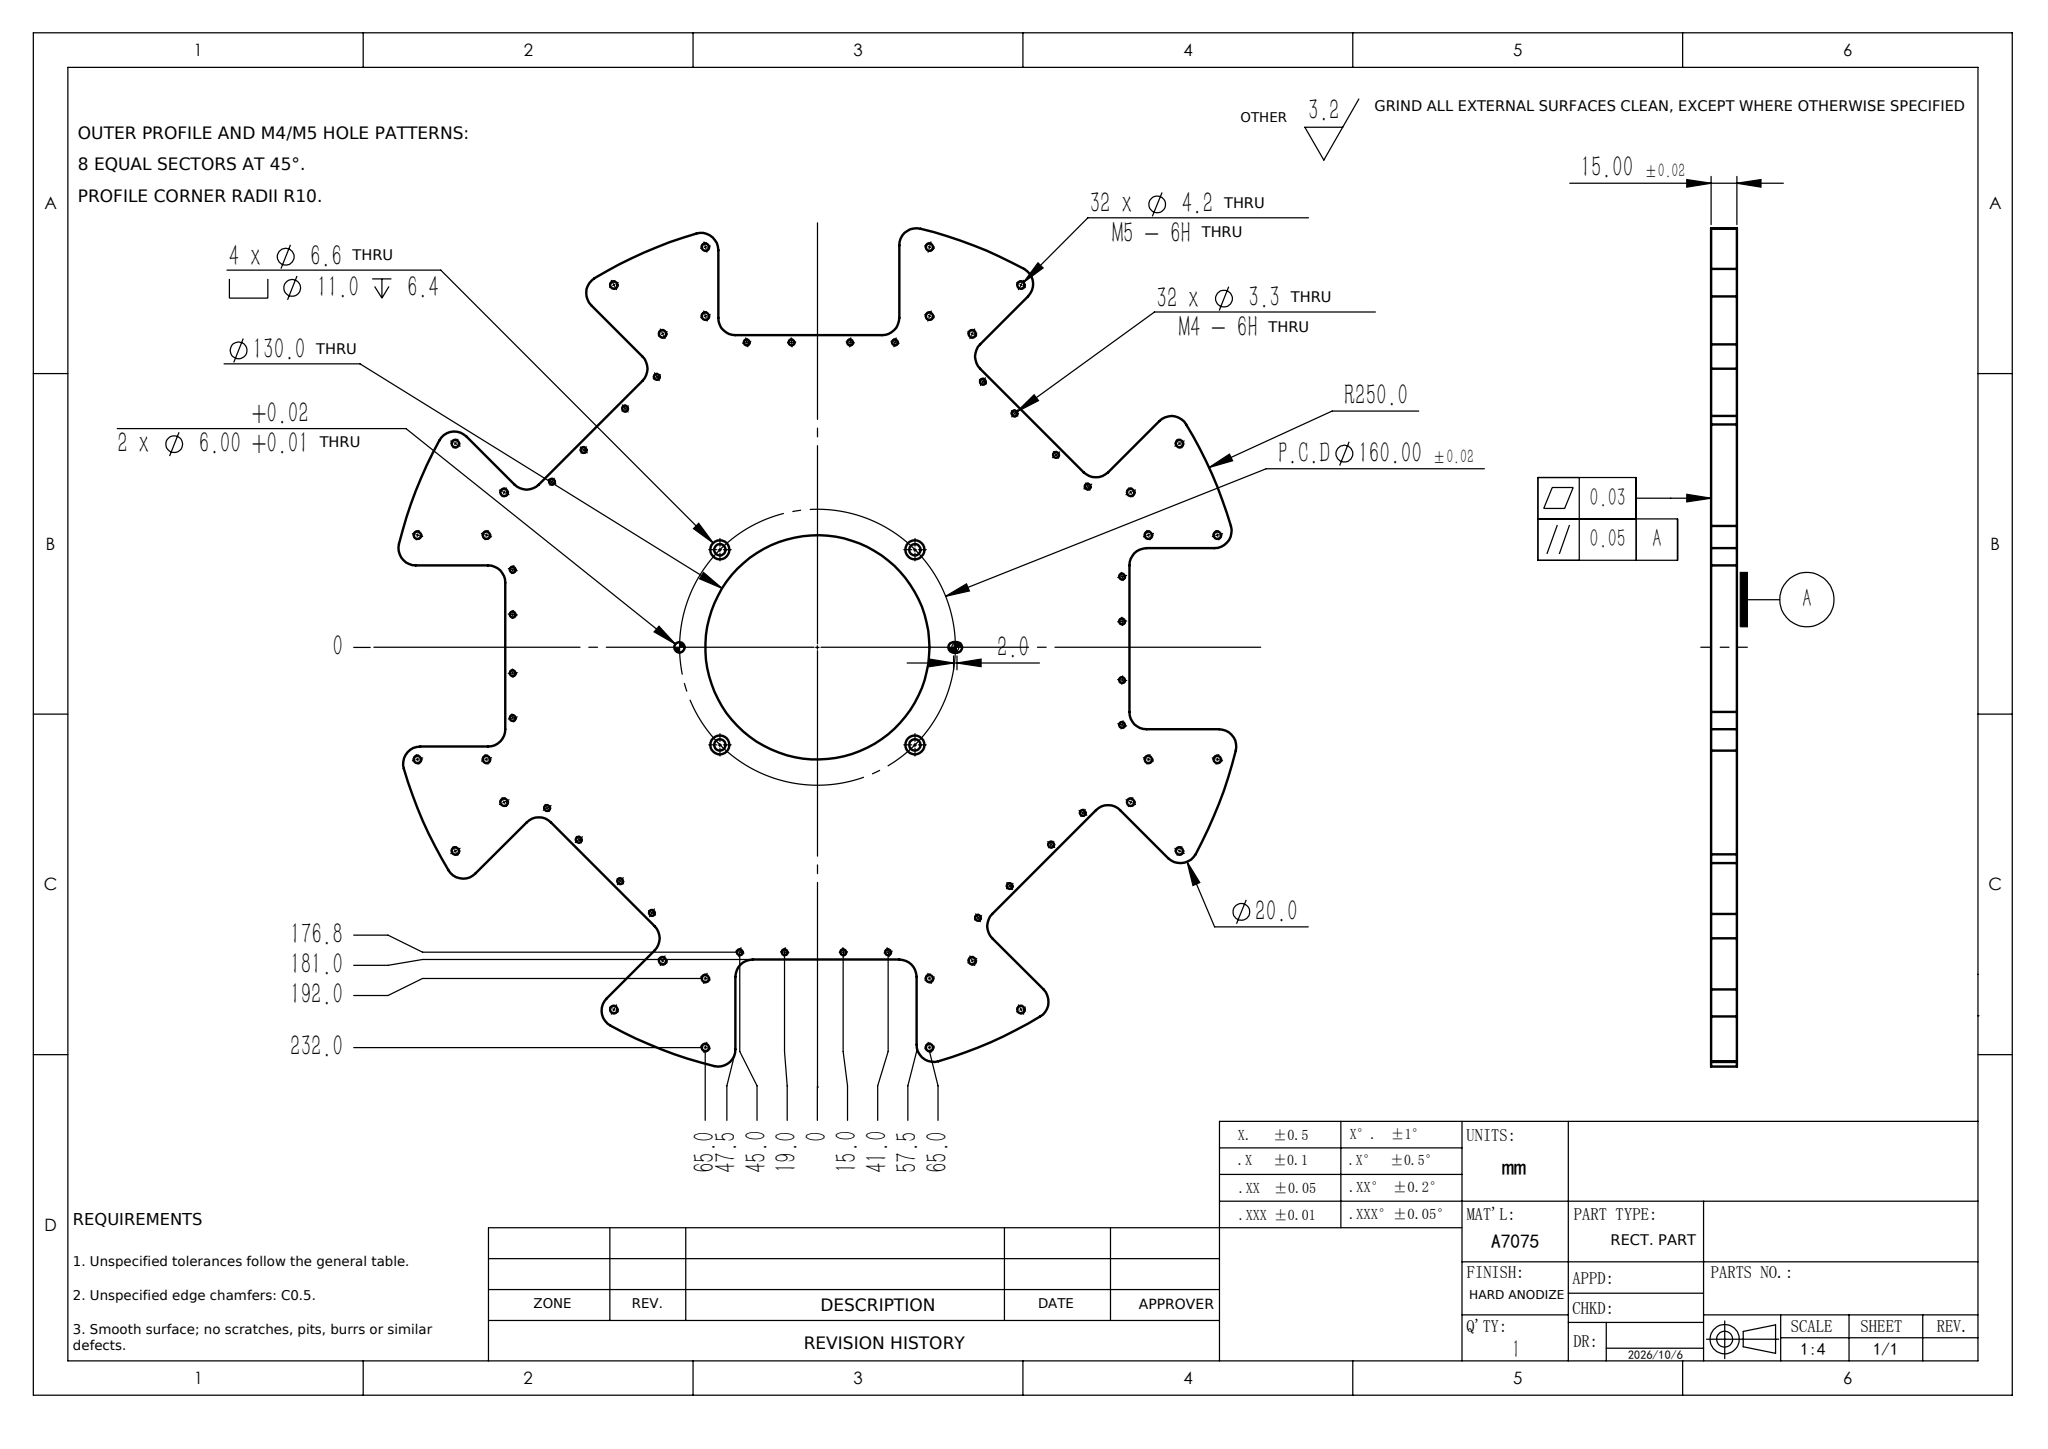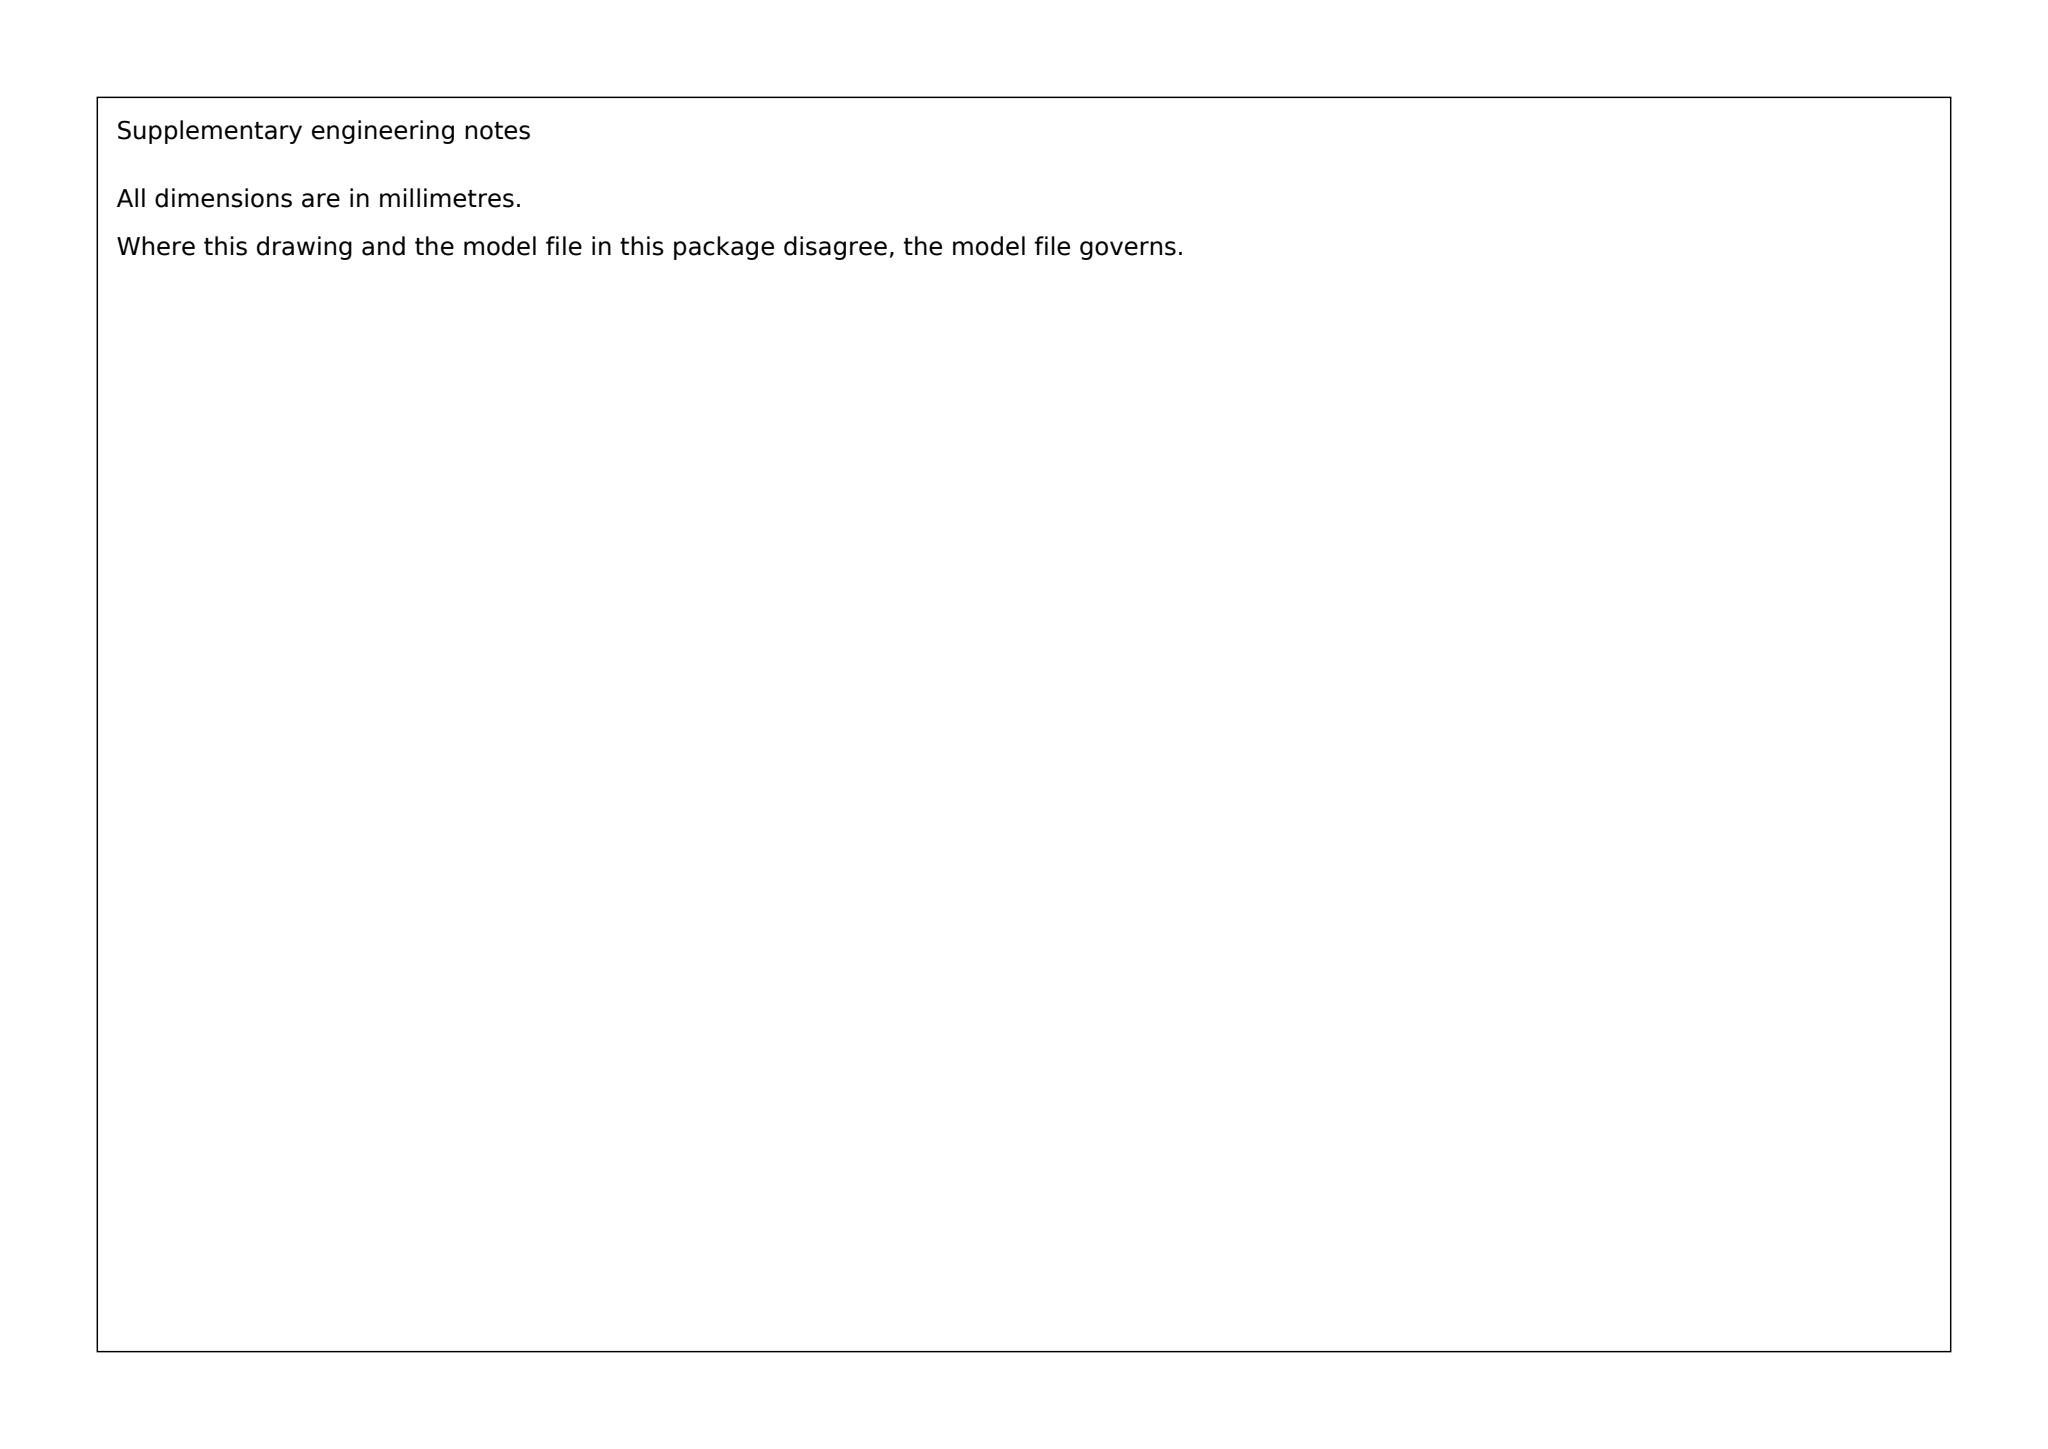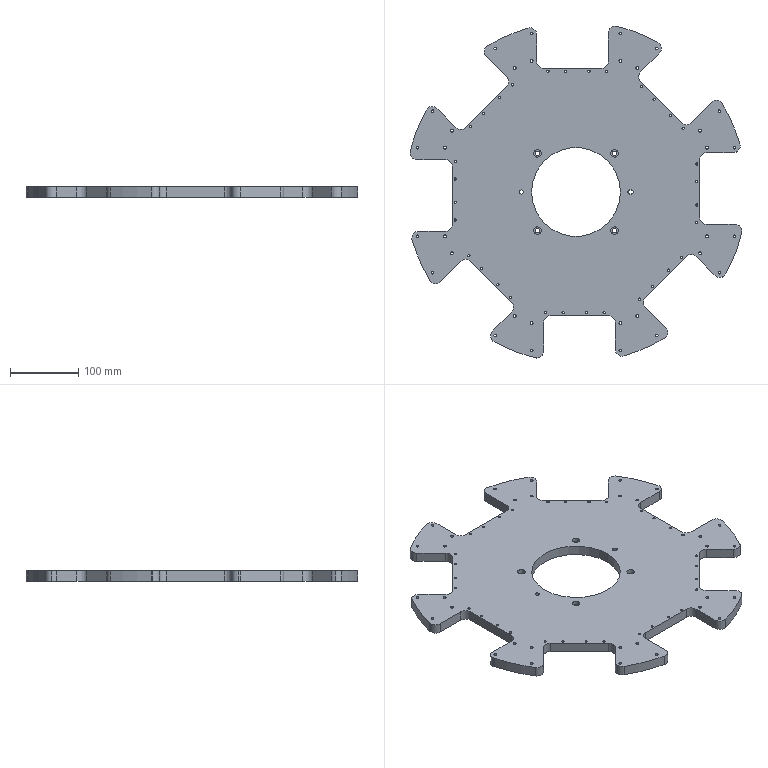Part | SolidWorks | mm | material A7075 | 1 solid | 229 faces | box 486.02 x 486.02 x 15 mm | volume 1881476 mm3 | cylinder 197 | plane 32 | commonest cylinder face diameters 3.3 x64 4.2 x64 20 x38 11 x8 6.6 x8 500 x8 6 x5 130 x2